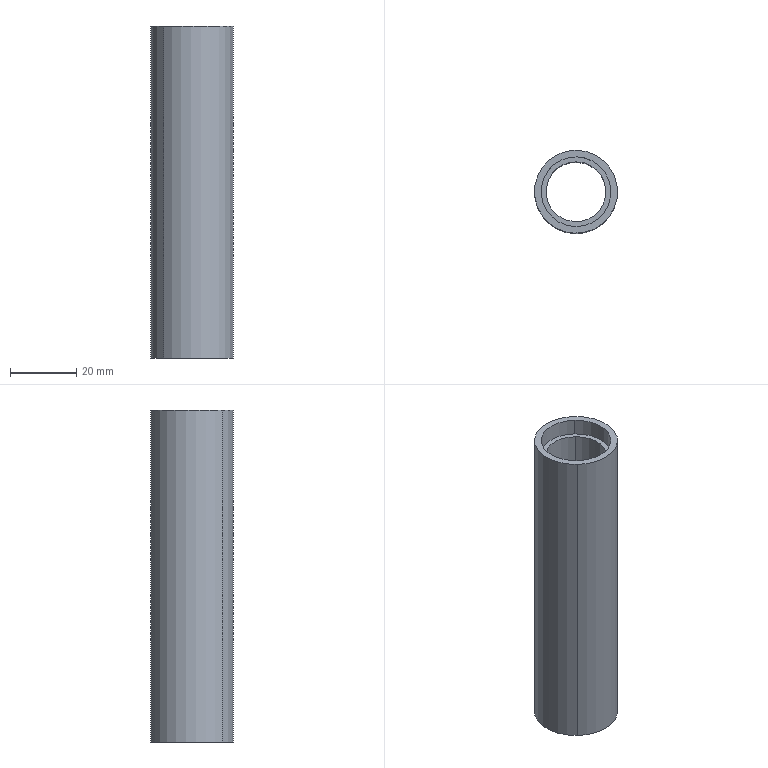Component | SolidWorks | GuideWheelAssembly2-1_Roller1-1 | 1 solid | 12 faces | box 25 x 25 x 100 mm | volume 22722 mm3 | cylinder 8 | plane 4 | commonest cylinder face diameters 21 x4 18 x2 25 x2
build123d program:
from build123d import *


with BuildPart() as part:
    # Sketch1 → Revolve1 (revolve)
    with BuildSketch(Plane.XY, mode=Mode.PRIVATE) as revolve1_sk:
        Polygon((0, 10.5), (5, 10.5), (5, 9), (95, 9), (95, 10.5), (100, 10.5), (100, 12.5), (0, 12.5), align=None)
    revolve(revolve1_sk.sketch.rotate(Axis((-1300.924, 0, 0), (1, 0, 0)), 90), axis=Axis((-1300.924, 0, 0), (1, 0, 0)))


solid = part.part

# Placed as in the assembly
solid = solid.moved(Location((-479.97, -65, 117), (0, 90, 0)))
STEP:
#1=CARTESIAN_POINT('',(-18.613,-2.258,4.409));
#2=VERTEX_POINT('',#1);
#3=CARTESIAN_POINT('',(-19.18,-2.86,4.409));
#4=VERTEX_POINT('',#3);
#5=CARTESIAN_POINT('',(-18.896,-2.559,4.409));
#6=DIRECTION('',(-0.,-0.,1.));
#7=DIRECTION('',(-0.686,-0.7276,0.));
#8=AXIS2_PLACEMENT_3D('',#5,#6,#7);
#9=CIRCLE('',#8,0.4134);
#10=EDGE_CURVE('',#2,#4,#9,.T.);
#11=ORIENTED_EDGE('',*,*,#10,.F.);
#12=CARTESIAN_POINT('',(-18.613,-2.258,4.606));
#13=VERTEX_POINT('',#12);
#14=CARTESIAN_POINT('',(-18.613,-2.258,55.824));
#15=DIRECTION('',(-0.,-0.,1.));
#16=VECTOR('',#15,39.37);
#17=LINE('',#14,#16);
#18=EDGE_CURVE('',#2,#13,#17,.T.);
#19=ORIENTED_EDGE('',*,*,#18,.T.);
#20=CARTESIAN_POINT('',(-19.18,-2.86,4.606));
#21=VERTEX_POINT('',#20);
#22=CARTESIAN_POINT('',(-18.896,-2.559,4.606));
#23=DIRECTION('',(-0.,-0.,1.));
#24=DIRECTION('',(-0.686,-0.7276,0.));
#25=AXIS2_PLACEMENT_3D('',#22,#23,#24);
#26=CIRCLE('',#25,0.4134);
#27=EDGE_CURVE('',#13,#21,#26,.T.);
#28=ORIENTED_EDGE('',*,*,#27,.T.);
#29=CARTESIAN_POINT('',(-19.18,-2.86,55.824));
#30=DIRECTION('',(-0.,-0.,1.));
#31=VECTOR('',#30,39.37);
#32=LINE('',#29,#31);
#33=EDGE_CURVE('',#4,#21,#32,.T.);
#34=ORIENTED_EDGE('',*,*,#33,.F.);
#35=EDGE_LOOP('',(#11,#19,#28,#34));
#36=FACE_OUTER_BOUND('',#35,.T.);
#37=CARTESIAN_POINT('',(-18.896,-2.559,55.824));
#38=DIRECTION('',(-0.,-0.,1.));
#39=DIRECTION('',(-0.686,-0.7276,0.));
#40=AXIS2_PLACEMENT_3D('',#37,#38,#39);
#41=CYLINDRICAL_SURFACE('',#40,0.4134);
#42=ADVANCED_FACE('',(#36),#41,.F.);
#43=CARTESIAN_POINT('',(-18.653,-2.301,0.8661));
#44=VERTEX_POINT('',#43);
#45=CARTESIAN_POINT('',(-19.14,-2.817,0.8661));
#46=VERTEX_POINT('',#45);
#47=CARTESIAN_POINT('',(-18.896,-2.559,0.8661));
#48=DIRECTION('',(-0.,-0.,1.));
#49=DIRECTION('',(-0.686,-0.7276,-0.));
#50=AXIS2_PLACEMENT_3D('',#47,#48,#49);
#51=CIRCLE('',#50,0.3543);
#52=EDGE_CURVE('',#44,#46,#51,.T.);
#53=ORIENTED_EDGE('',*,*,#52,.F.);
#54=CARTESIAN_POINT('',(-18.653,-2.301,4.409));
#55=VERTEX_POINT('',#54);
#56=CARTESIAN_POINT('',(-18.653,-2.301,55.824));
#57=DIRECTION('',(-0.,-0.,1.));
#58=VECTOR('',#57,39.37);
#59=LINE('',#56,#58);
#60=EDGE_CURVE('',#44,#55,#59,.T.);
#61=ORIENTED_EDGE('',*,*,#60,.T.);
#62=CARTESIAN_POINT('',(-19.14,-2.817,4.409));
#63=VERTEX_POINT('',#62);
#64=CARTESIAN_POINT('',(-18.896,-2.559,4.409));
#65=DIRECTION('',(-0.,-0.,1.));
#66=DIRECTION('',(-0.686,-0.7276,0.));
#67=AXIS2_PLACEMENT_3D('',#64,#65,#66);
#68=CIRCLE('',#67,0.3543);
#69=EDGE_CURVE('',#55,#63,#68,.T.);
#70=ORIENTED_EDGE('',*,*,#69,.T.);
#71=CARTESIAN_POINT('',(-19.14,-2.817,55.824));
#72=DIRECTION('',(-0.,-0.,1.));
#73=VECTOR('',#72,39.37);
#74=LINE('',#71,#73);
#75=EDGE_CURVE('',#46,#63,#74,.T.);
#76=ORIENTED_EDGE('',*,*,#75,.F.);
#77=EDGE_LOOP('',(#53,#61,#70,#76));
#78=FACE_OUTER_BOUND('',#77,.T.);
#79=CARTESIAN_POINT('',(-18.896,-2.559,55.824));
#80=DIRECTION('',(-0.,-0.,1.));
#81=DIRECTION('',(-0.686,-0.7276,0.));
#82=AXIS2_PLACEMENT_3D('',#79,#80,#81);
#83=CYLINDRICAL_SURFACE('',#82,0.3543);
#84=ADVANCED_FACE('',(#78),#83,.F.);
#85=CARTESIAN_POINT('',(-18.613,-2.258,0.6693));
#86=VERTEX_POINT('',#85);
#87=CARTESIAN_POINT('',(-19.18,-2.86,0.6693));
#88=VERTEX_POINT('',#87);
#89=CARTESIAN_POINT('',(-18.896,-2.559,0.6693));
#90=DIRECTION('',(-0.,-0.,1.));
#91=DIRECTION('',(-0.686,-0.7276,-0.));
#92=AXIS2_PLACEMENT_3D('',#89,#90,#91);
#93=CIRCLE('',#92,0.4134);
#94=EDGE_CURVE('',#86,#88,#93,.T.);
#95=ORIENTED_EDGE('',*,*,#94,.F.);
#96=CARTESIAN_POINT('',(-18.613,-2.258,0.8661));
#97=VERTEX_POINT('',#96);
#98=CARTESIAN_POINT('',(-18.613,-2.258,55.824));
#99=DIRECTION('',(-0.,-0.,1.));
#100=VECTOR('',#99,39.37);
#101=LINE('',#98,#100);
#102=EDGE_CURVE('',#86,#97,#101,.T.);
#103=ORIENTED_EDGE('',*,*,#102,.T.);
#104=CARTESIAN_POINT('',(-19.18,-2.86,0.8661));
#105=VERTEX_POINT('',#104);
#106=CARTESIAN_POINT('',(-18.896,-2.559,0.8661));
#107=DIRECTION('',(-0.,-0.,1.));
#108=DIRECTION('',(-0.686,-0.7276,-0.));
#109=AXIS2_PLACEMENT_3D('',#106,#107,#108);
#110=CIRCLE('',#109,0.4134);
#111=EDGE_CURVE('',#97,#105,#110,.T.);
#112=ORIENTED_EDGE('',*,*,#111,.T.);
#113=CARTESIAN_POINT('',(-19.18,-2.86,55.824));
#114=DIRECTION('',(-0.,-0.,1.));
#115=VECTOR('',#114,39.37);
#116=LINE('',#113,#115);
#117=EDGE_CURVE('',#88,#105,#116,.T.);
#118=ORIENTED_EDGE('',*,*,#117,.F.);
#119=EDGE_LOOP('',(#95,#103,#112,#118));
#120=FACE_OUTER_BOUND('',#119,.T.);
#121=CARTESIAN_POINT('',(-18.896,-2.559,55.824));
#122=DIRECTION('',(-0.,-0.,1.));
#123=DIRECTION('',(-0.686,-0.7276,0.));
#124=AXIS2_PLACEMENT_3D('',#121,#122,#123);
#125=CYLINDRICAL_SURFACE('',#124,0.4134);
#126=ADVANCED_FACE('',(#120),#125,.F.);
#127=CARTESIAN_POINT('',(-19.234,-2.917,0.6693));
#128=VERTEX_POINT('',#127);
#129=CARTESIAN_POINT('',(-18.559,-2.201,0.6693));
#130=VERTEX_POINT('',#129);
#131=CARTESIAN_POINT('',(-18.896,-2.559,0.6693));
#132=DIRECTION('',(-0.,-0.,1.));
#133=DIRECTION('',(-0.686,-0.7276,-0.));
#134=AXIS2_PLACEMENT_3D('',#131,#132,#133);
#135=CIRCLE('',#134,0.4921);
#136=EDGE_CURVE('',#128,#130,#135,.T.);
#137=ORIENTED_EDGE('',*,*,#136,.T.);
#138=CARTESIAN_POINT('',(-18.559,-2.201,4.606));
#139=VERTEX_POINT('',#138);
#140=CARTESIAN_POINT('',(-18.559,-2.201,55.824));
#141=DIRECTION('',(-0.,-0.,1.));
#142=VECTOR('',#141,39.37);
#143=LINE('',#140,#142);
#144=EDGE_CURVE('',#130,#139,#143,.T.);
#145=ORIENTED_EDGE('',*,*,#144,.T.);
#146=CARTESIAN_POINT('',(-19.234,-2.917,4.606));
#147=VERTEX_POINT('',#146);
#148=CARTESIAN_POINT('',(-18.896,-2.559,4.606));
#149=DIRECTION('',(-0.,-0.,1.));
#150=DIRECTION('',(-0.686,-0.7276,0.));
#151=AXIS2_PLACEMENT_3D('',#148,#149,#150);
#152=CIRCLE('',#151,0.4921);
#153=EDGE_CURVE('',#147,#139,#152,.T.);
#154=ORIENTED_EDGE('',*,*,#153,.F.);
#155=CARTESIAN_POINT('',(-19.234,-2.917,55.824));
#156=DIRECTION('',(-0.,-0.,1.));
#157=VECTOR('',#156,39.37);
#158=LINE('',#155,#157);
#159=EDGE_CURVE('',#128,#147,#158,.T.);
#160=ORIENTED_EDGE('',*,*,#159,.F.);
#161=EDGE_LOOP('',(#137,#145,#154,#160));
#162=FACE_OUTER_BOUND('',#161,.T.);
#163=CARTESIAN_POINT('',(-18.896,-2.559,55.824));
#164=DIRECTION('',(-0.,-0.,1.));
#165=DIRECTION('',(-0.686,-0.7276,0.));
#166=AXIS2_PLACEMENT_3D('',#163,#164,#165);
#167=CYLINDRICAL_SURFACE('',#166,0.4921);
#168=ADVANCED_FACE('',(#162),#167,.T.);
#169=CARTESIAN_POINT('',(-18.896,-2.559,4.606));
#170=DIRECTION('',(-0.,-0.,1.));
#171=DIRECTION('',(-0.686,-0.7276,0.));
#172=AXIS2_PLACEMENT_3D('',#169,#170,#171);
#173=CIRCLE('',#172,0.4134);
#174=EDGE_CURVE('',#21,#13,#173,.T.);
#175=ORIENTED_EDGE('',*,*,#174,.F.);
#176=ORIENTED_EDGE('',*,*,#27,.F.);
#177=EDGE_LOOP('',(#175,#176));
#178=FACE_BOUND('',#177,.T.);
#179=ORIENTED_EDGE('',*,*,#153,.T.);
#180=CARTESIAN_POINT('',(-18.896,-2.559,4.606));
#181=DIRECTION('',(-0.,-0.,1.));
#182=DIRECTION('',(-0.686,-0.7276,0.));
#183=AXIS2_PLACEMENT_3D('',#180,#181,#182);
#184=CIRCLE('',#183,0.4921);
#185=EDGE_CURVE('',#139,#147,#184,.T.);
#186=ORIENTED_EDGE('',*,*,#185,.T.);
#187=EDGE_LOOP('',(#179,#186));
#188=FACE_OUTER_BOUND('',#187,.T.);
#189=CARTESIAN_POINT('',(-18.596,-2.843,4.606));
#190=DIRECTION('',(0.,0.,-1.));
#191=DIRECTION('',(0.686,0.7276,0.));
#192=AXIS2_PLACEMENT_3D('',#189,#190,#191);
#193=PLANE('',#192);
#194=ADVANCED_FACE('',(#178,#188),#193,.F.);
#195=ORIENTED_EDGE('',*,*,#144,.F.);
#196=CARTESIAN_POINT('',(-18.896,-2.559,0.6693));
#197=DIRECTION('',(-0.,-0.,1.));
#198=DIRECTION('',(-0.686,-0.7276,-0.));
#199=AXIS2_PLACEMENT_3D('',#196,#197,#198);
#200=CIRCLE('',#199,0.4921);
#201=EDGE_CURVE('',#130,#128,#200,.T.);
#202=ORIENTED_EDGE('',*,*,#201,.T.);
#203=ORIENTED_EDGE('',*,*,#159,.T.);
#204=ORIENTED_EDGE('',*,*,#185,.F.);
#205=EDGE_LOOP('',(#195,#202,#203,#204));
#206=FACE_OUTER_BOUND('',#205,.T.);
#207=CARTESIAN_POINT('',(-18.896,-2.559,55.824));
#208=DIRECTION('',(-0.,-0.,1.));
#209=DIRECTION('',(-0.686,-0.7276,0.));
#210=AXIS2_PLACEMENT_3D('',#207,#208,#209);
#211=CYLINDRICAL_SURFACE('',#210,0.4921);
#212=ADVANCED_FACE('',(#206),#211,.T.);
#213=ORIENTED_EDGE('',*,*,#136,.F.);
#214=ORIENTED_EDGE('',*,*,#201,.F.);
#215=EDGE_LOOP('',(#213,#214));
#216=FACE_OUTER_BOUND('',#215,.T.);
#217=CARTESIAN_POINT('',(-18.896,-2.559,0.6693));
#218=DIRECTION('',(-0.,-0.,1.));
#219=DIRECTION('',(-0.686,-0.7276,-0.));
#220=AXIS2_PLACEMENT_3D('',#217,#218,#219);
#221=CIRCLE('',#220,0.4134);
#222=EDGE_CURVE('',#88,#86,#221,.T.);
#223=ORIENTED_EDGE('',*,*,#222,.T.);
#224=ORIENTED_EDGE('',*,*,#94,.T.);
#225=EDGE_LOOP('',(#223,#224));
#226=FACE_BOUND('',#225,.T.);
#227=CARTESIAN_POINT('',(-18.538,-2.897,0.6693));
#228=DIRECTION('',(-0.,-0.,1.));
#229=DIRECTION('',(-0.686,-0.7276,-0.));
#230=AXIS2_PLACEMENT_3D('',#227,#228,#229);
#231=PLANE('',#230);
#232=ADVANCED_FACE('',(#216,#226),#231,.F.);
#233=ORIENTED_EDGE('',*,*,#102,.F.);
#234=ORIENTED_EDGE('',*,*,#222,.F.);
#235=ORIENTED_EDGE('',*,*,#117,.T.);
#236=CARTESIAN_POINT('',(-18.896,-2.559,0.8661));
#237=DIRECTION('',(-0.,-0.,1.));
#238=DIRECTION('',(-0.686,-0.7276,-0.));
#239=AXIS2_PLACEMENT_3D('',#236,#237,#238);
#240=CIRCLE('',#239,0.4134);
#241=EDGE_CURVE('',#105,#97,#240,.T.);
#242=ORIENTED_EDGE('',*,*,#241,.T.);
#243=EDGE_LOOP('',(#233,#234,#235,#242));
#244=FACE_OUTER_BOUND('',#243,.T.);
#245=CARTESIAN_POINT('',(-18.896,-2.559,55.824));
#246=DIRECTION('',(-0.,-0.,1.));
#247=DIRECTION('',(-0.686,-0.7276,0.));
#248=AXIS2_PLACEMENT_3D('',#245,#246,#247);
#249=CYLINDRICAL_SURFACE('',#248,0.4134);
#250=ADVANCED_FACE('',(#244),#249,.F.);
#251=ORIENTED_EDGE('',*,*,#241,.F.);
#252=ORIENTED_EDGE('',*,*,#111,.F.);
#253=EDGE_LOOP('',(#251,#252));
#254=FACE_OUTER_BOUND('',#253,.T.);
#255=CARTESIAN_POINT('',(-18.896,-2.559,0.8661));
#256=DIRECTION('',(-0.,-0.,1.));
#257=DIRECTION('',(-0.686,-0.7276,-0.));
#258=AXIS2_PLACEMENT_3D('',#255,#256,#257);
#259=CIRCLE('',#258,0.3543);
#260=EDGE_CURVE('',#46,#44,#259,.T.);
#261=ORIENTED_EDGE('',*,*,#260,.T.);
#262=ORIENTED_EDGE('',*,*,#52,.T.);
#263=EDGE_LOOP('',(#261,#262));
#264=FACE_BOUND('',#263,.T.);
#265=CARTESIAN_POINT('',(-18.639,-2.802,0.8661));
#266=DIRECTION('',(-0.,-0.,1.));
#267=DIRECTION('',(-0.686,-0.7276,-0.));
#268=AXIS2_PLACEMENT_3D('',#265,#266,#267);
#269=PLANE('',#268);
#270=ADVANCED_FACE('',(#254,#264),#269,.F.);
#271=ORIENTED_EDGE('',*,*,#60,.F.);
#272=ORIENTED_EDGE('',*,*,#260,.F.);
#273=ORIENTED_EDGE('',*,*,#75,.T.);
#274=CARTESIAN_POINT('',(-18.896,-2.559,4.409));
#275=DIRECTION('',(-0.,-0.,1.));
#276=DIRECTION('',(-0.686,-0.7276,0.));
#277=AXIS2_PLACEMENT_3D('',#274,#275,#276);
#278=CIRCLE('',#277,0.3543);
#279=EDGE_CURVE('',#63,#55,#278,.T.);
#280=ORIENTED_EDGE('',*,*,#279,.T.);
#281=EDGE_LOOP('',(#271,#272,#273,#280));
#282=FACE_OUTER_BOUND('',#281,.T.);
#283=CARTESIAN_POINT('',(-18.896,-2.559,55.824));
#284=DIRECTION('',(-0.,-0.,1.));
#285=DIRECTION('',(-0.686,-0.7276,0.));
#286=AXIS2_PLACEMENT_3D('',#283,#284,#285);
#287=CYLINDRICAL_SURFACE('',#286,0.3543);
#288=ADVANCED_FACE('',(#282),#287,.F.);
#289=ORIENTED_EDGE('',*,*,#279,.F.);
#290=ORIENTED_EDGE('',*,*,#69,.F.);
#291=EDGE_LOOP('',(#289,#290));
#292=FACE_BOUND('',#291,.T.);
#293=CARTESIAN_POINT('',(-18.896,-2.559,4.409));
#294=DIRECTION('',(-0.,-0.,1.));
#295=DIRECTION('',(-0.686,-0.7276,0.));
#296=AXIS2_PLACEMENT_3D('',#293,#294,#295);
#297=CIRCLE('',#296,0.4134);
#298=EDGE_CURVE('',#4,#2,#297,.T.);
#299=ORIENTED_EDGE('',*,*,#298,.T.);
#300=ORIENTED_EDGE('',*,*,#10,.T.);
#301=EDGE_LOOP('',(#299,#300));
#302=FACE_OUTER_BOUND('',#301,.T.);
#303=CARTESIAN_POINT('',(-18.596,-2.843,4.409));
#304=DIRECTION('',(0.,0.,-1.));
#305=DIRECTION('',(0.686,0.7276,0.));
#306=AXIS2_PLACEMENT_3D('',#303,#304,#305);
#307=PLANE('',#306);
#308=ADVANCED_FACE('',(#292,#302),#307,.F.);
#309=ORIENTED_EDGE('',*,*,#18,.F.);
#310=ORIENTED_EDGE('',*,*,#298,.F.);
#311=ORIENTED_EDGE('',*,*,#33,.T.);
#312=ORIENTED_EDGE('',*,*,#174,.T.);
#313=EDGE_LOOP('',(#309,#310,#311,#312));
#314=FACE_OUTER_BOUND('',#313,.T.);
#315=CARTESIAN_POINT('',(-18.896,-2.559,55.824));
#316=DIRECTION('',(-0.,-0.,1.));
#317=DIRECTION('',(-0.686,-0.7276,0.));
#318=AXIS2_PLACEMENT_3D('',#315,#316,#317);
#319=CYLINDRICAL_SURFACE('',#318,0.4134);
#320=ADVANCED_FACE('',(#314),#319,.F.);
#321=CLOSED_SHELL('',(#42,#84,#126,#168,#194,#212,#232,#250,#270,#288,#308,#320));
#322=MANIFOLD_SOLID_BREP('',#321);
#323=CARTESIAN_POINT('',(0.,0.,0.));
#324=DIRECTION('',(0.,0.,1.));
#325=DIRECTION('',(1.,0.,0.));
#326=AXIS2_PLACEMENT_3D('',#323,#324,#325);
#327=(LENGTH_UNIT()NAMED_UNIT(*)SI_UNIT($,.METRE.));
#328=LENGTH_MEASURE_WITH_UNIT(LENGTH_MEASURE(0.0254),#327);
#329=DIMENSIONAL_EXPONENTS(1.,0.,0.,0.,0.,0.,0.);
#330=(CONVERSION_BASED_UNIT('',#328)LENGTH_UNIT()NAMED_UNIT(#329));
#331=UNCERTAINTY_MEASURE_WITH_UNIT(LENGTH_MEASURE(0.00001),#330,'','');
#332=(NAMED_UNIT(*)PLANE_ANGLE_UNIT()SI_UNIT($,.RADIAN.));
#333=(NAMED_UNIT(*)SI_UNIT($,.STERADIAN.)SOLID_ANGLE_UNIT());
#334=(GEOMETRIC_REPRESENTATION_CONTEXT(3)GLOBAL_UNCERTAINTY_ASSIGNED_CONTEXT((#331))GLOBAL_UNIT_ASSIGNED_CONTEXT((#330,#332,#333))REPRESENTATION_CONTEXT('',''));
#335=ADVANCED_BREP_SHAPE_REPRESENTATION('',(#322,#326),#334);
#336=COLOUR_RGB('',0.7922,0.8196,0.9333);
#337=FILL_AREA_STYLE_COLOUR('',#336);
#338=FILL_AREA_STYLE('',(#337));
#339=SURFACE_STYLE_FILL_AREA(#338);
#340=SURFACE_SIDE_STYLE('',(#339));
#341=SURFACE_STYLE_USAGE(.BOTH.,#340);
#342=PRESENTATION_STYLE_ASSIGNMENT((#341));
#343=STYLED_ITEM('',(#342),#322);
#344=PRESENTATION_LAYER_ASSIGNMENT('','',(#343));
#345=(LENGTH_UNIT()NAMED_UNIT(*)SI_UNIT($,.METRE.));
#346=LENGTH_MEASURE_WITH_UNIT(LENGTH_MEASURE(0.0254),#345);
#347=DIMENSIONAL_EXPONENTS(1.,0.,0.,0.,0.,0.,0.);
#348=(CONVERSION_BASED_UNIT('',#346)LENGTH_UNIT()NAMED_UNIT(#347));
#349=UNCERTAINTY_MEASURE_WITH_UNIT(LENGTH_MEASURE(0.00001),#348,'','');
#350=(NAMED_UNIT(*)PLANE_ANGLE_UNIT()SI_UNIT($,.RADIAN.));
#351=(NAMED_UNIT(*)SI_UNIT($,.STERADIAN.)SOLID_ANGLE_UNIT());
#352=(GEOMETRIC_REPRESENTATION_CONTEXT(3)GLOBAL_UNCERTAINTY_ASSIGNED_CONTEXT((#349))GLOBAL_UNIT_ASSIGNED_CONTEXT((#348,#350,#351))REPRESENTATION_CONTEXT('',''));
#353=MECHANICAL_DESIGN_GEOMETRIC_PRESENTATION_REPRESENTATION('',(#343),#352);